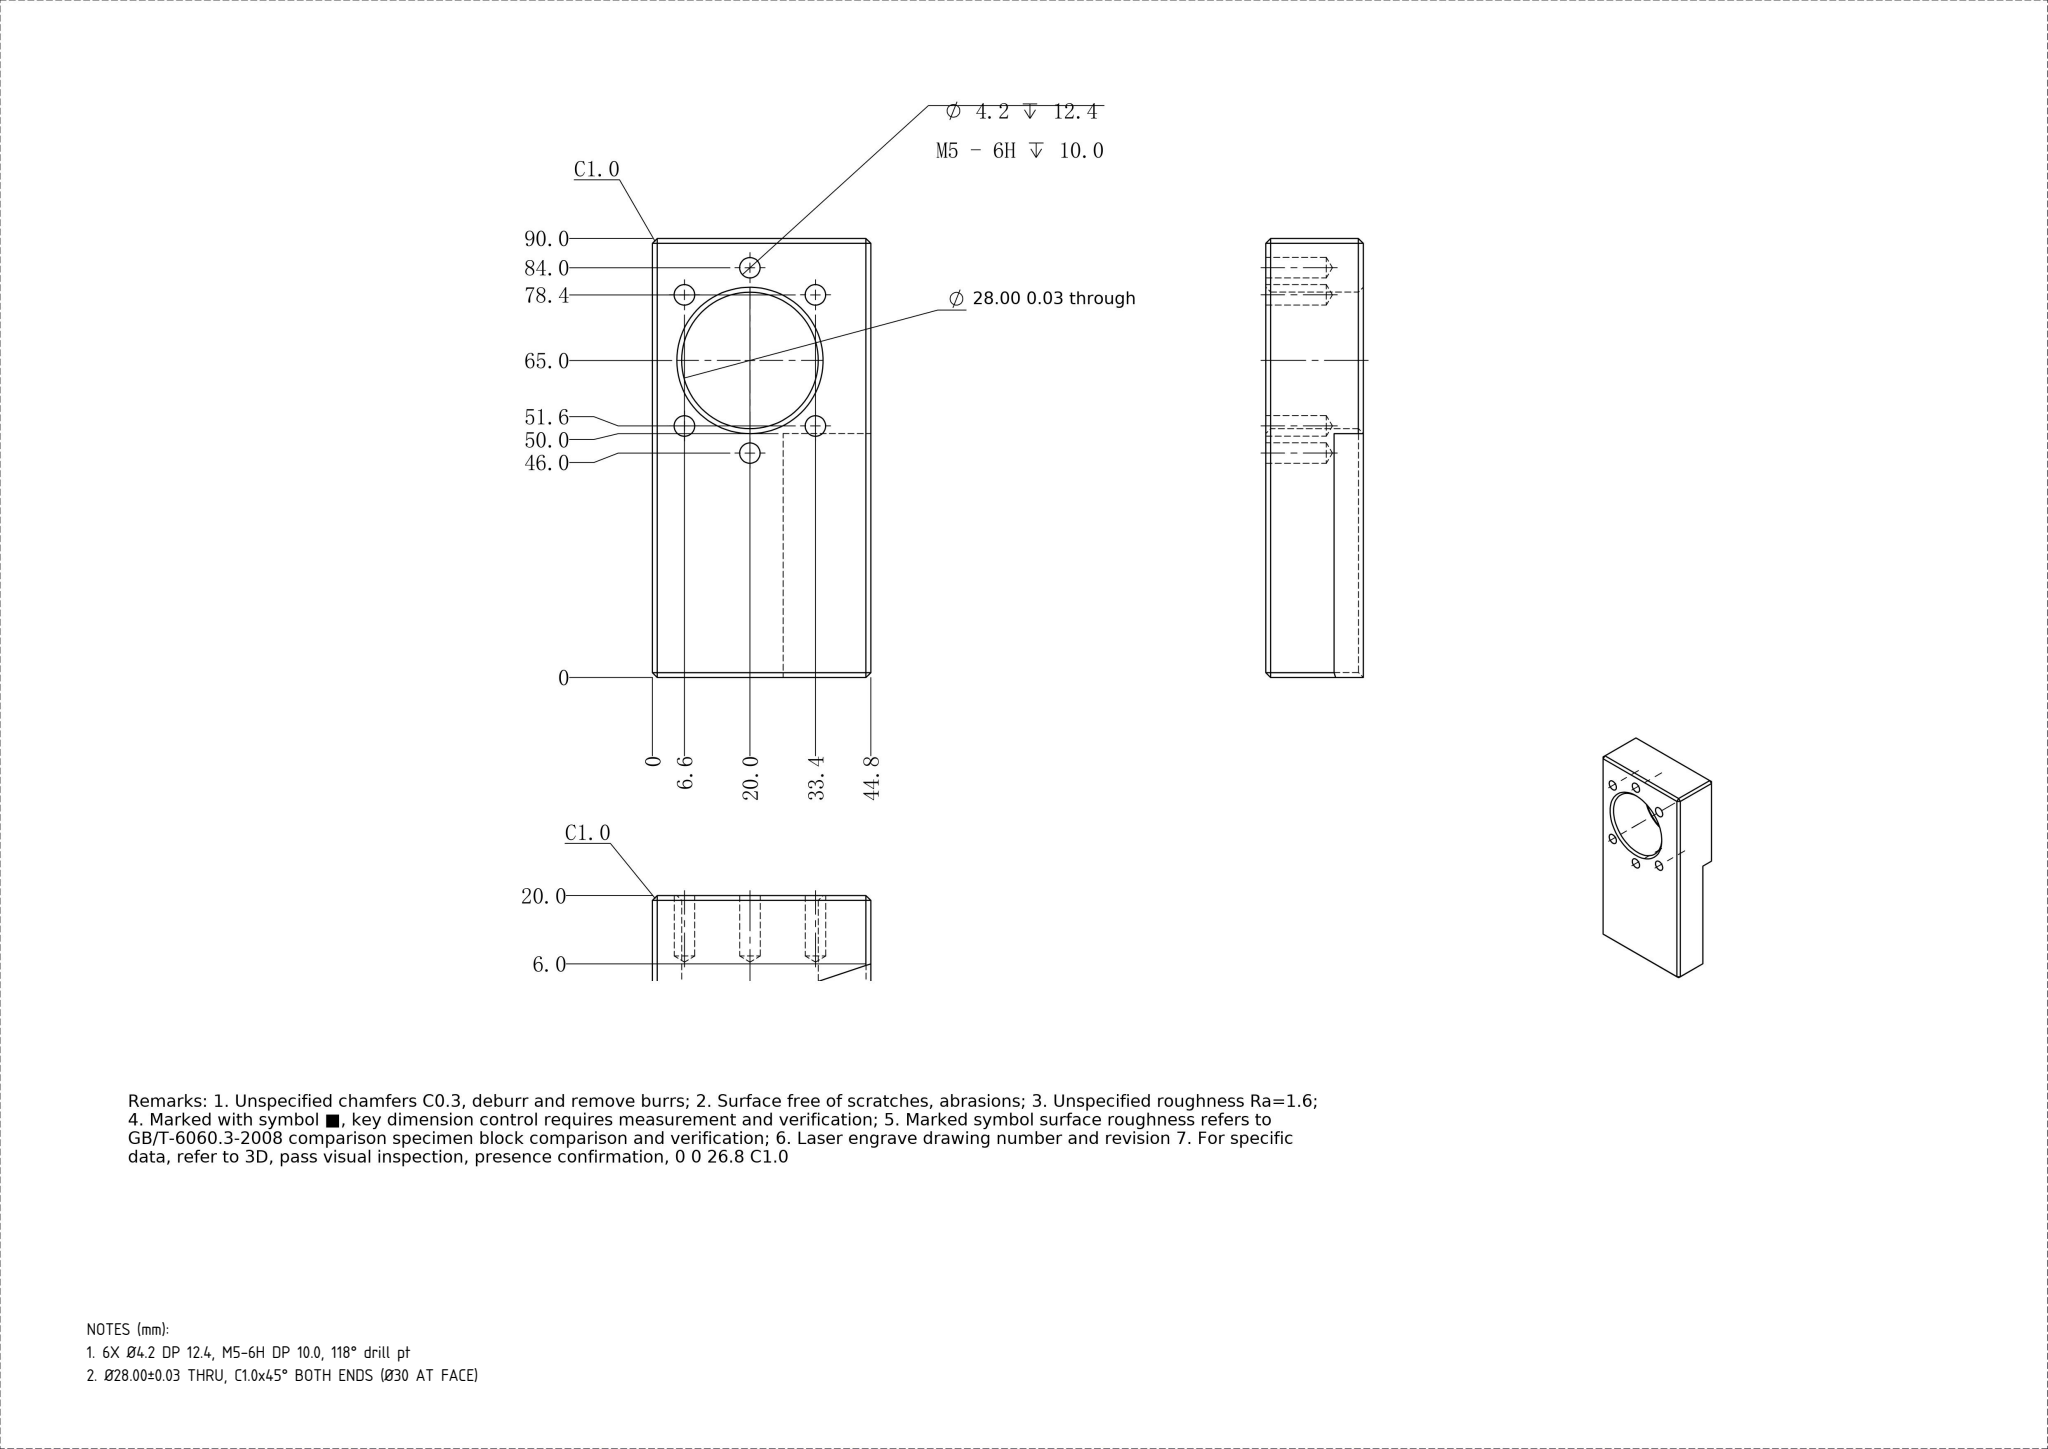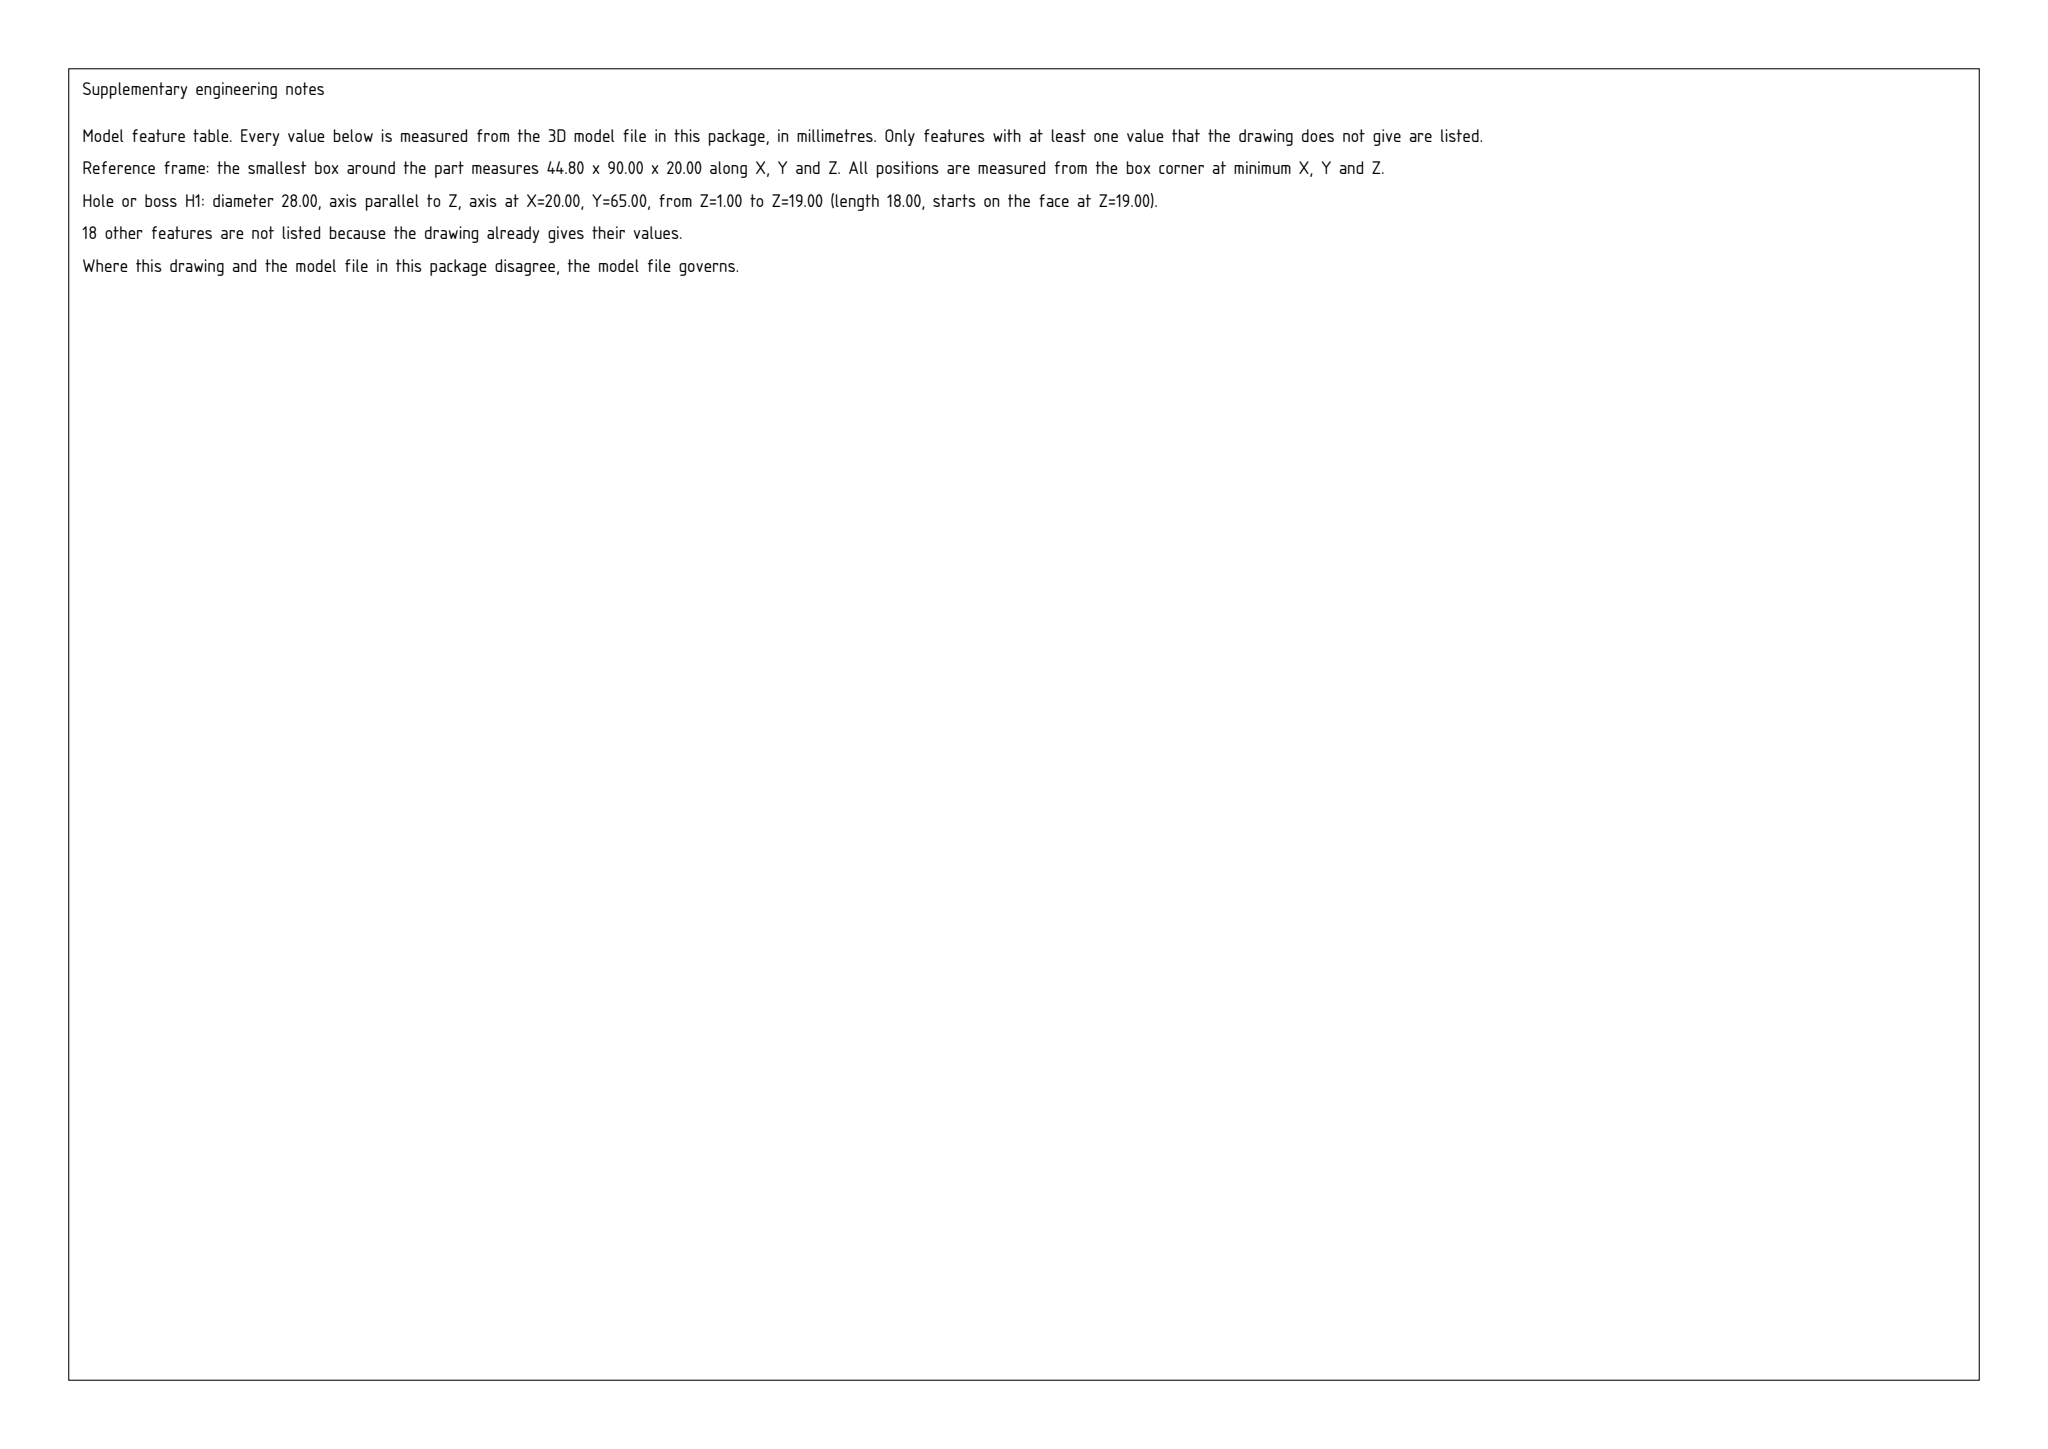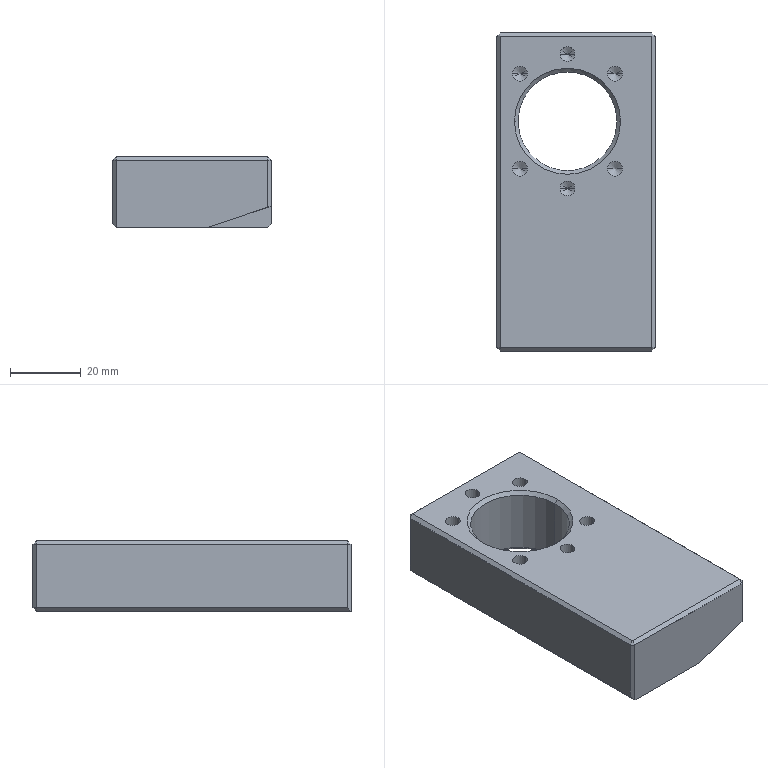Part | SolidWorks | mm | 1 solid | 55 faces | box 44.8 x 90 x 20 mm | volume 64214 mm3 | plane 25 | cone 16 | cylinder 14 | commonest cylinder face diameters 4.2 x12 28 x2
Drawing notes:
6X Ø4.2 DP 12.4, M5-6H DP 10.0, 118° drill pt | from the solid: Six Ø4.2 z-axis cyl L=12.4 at (6.56,51.56)(6.56,78.44)(20,46)(20,84)(33.44,51.56)(33.44,78.44); cones 118° ref dia 4.2
Ø28.00±0.03 THRU, C1.0x45° BOTH ENDS (Ø30 AT FACE) | from the solid: Ø28 bore L=18.0 in 20.0 thk plate; 2 cones 90° incl, ref dia 30.0/28.0 at each face
build123d program:
from build123d import *

# Parameters (mm, degrees)
SKETCH1_W             = 44.8
SKETCH1_H             = 20
BOSS_EXTRUDE1_DEPTH   = 25
SKETCH2_R             = 14
CUT_EXTRUDE1_DEPTH    = 40.074
M5_TAPPED_HOLE1_D     = 4.2
M5_TAPPED_HOLE1_DEPTH = 12.4
M5_TAPPED_HOLE1_TIP   = 1.262
MOVE_FACE1_BY         = 40
CUT_EXTRUDE2_DEPTH    = 50
CHAMFER1_SIZE         = 1


with BuildPart() as part:
    # Sketch1 → Boss-Extrude1 (new, symmetric)
    with BuildSketch(Plane(origin=(0, 0, 0), x_dir=(1, 0, 0), z_dir=(0, 1, 0))):
        Rectangle(SKETCH1_W, SKETCH1_H)
    extrude(amount=BOSS_EXTRUDE1_DEPTH, both=True)

    # Sketch2 → Cut-Extrude1 (cut, through all)
    with BuildSketch(Plane(origin=(0, 0, -10), x_dir=(-1, 0, 0), z_dir=(0, 0, -1))):
        with Locations((2.4, 0)):
            Circle(SKETCH2_R)
    extrude(amount=-CUT_EXTRUDE1_DEPTH, mode=Mode.SUBTRACT)

    # M5 Tapped Hole1
    with Locations(Plane.XY.offset(10)):
        with Locations((-15.835, -13.435), (-2.4, -19), (11.035, -13.435), (11.035, 13.435), (-2.4, 19), (-15.835, 13.435)):
            Hole(M5_TAPPED_HOLE1_D / 2, depth=M5_TAPPED_HOLE1_DEPTH)
            with Locations((0, 0, -(M5_TAPPED_HOLE1_DEPTH + M5_TAPPED_HOLE1_TIP / 2))):  # 118° drill point
                Cone(0, M5_TAPPED_HOLE1_D / 2, M5_TAPPED_HOLE1_TIP, mode=Mode.SUBTRACT)

    # Move Face1: a face moved outward by 40.0
    extrude(part.faces().sort_by_distance((0, -25, 0))[0], amount=MOVE_FACE1_BY, dir=(0, -1, 0))

    # Sketch5 → Cut-Extrude2 (cut)
    with BuildSketch(Plane.XZ.offset(65)):
        Polygon((22.4, -4), (4.4, -10), (22.4, -10), align=None)
    extrude(amount=-CUT_EXTRUDE2_DEPTH, mode=Mode.SUBTRACT)

    # Chamfer1
    chamfer1_edges = [part.edges().sort_by_distance(p)[0] for p in [
        (-22.4, 25, 0),
        (11.6, 0, 10),
        (11.6, 0, -10),
        (0, 25, 10),
        (22.4, 25, 0),
        (0, -65, 10),
        (-22.4, -65, 0),
        (22.4, -65, 3),
        (22.4, -20, 10),
        (-22.4, -20, 10),
        (-22.4, -20, -10),
        (22.4, 5, -10),
        (0, 25, -10),
    ]]
    chamfer(chamfer1_edges, length=CHAMFER1_SIZE)


solid = part.part